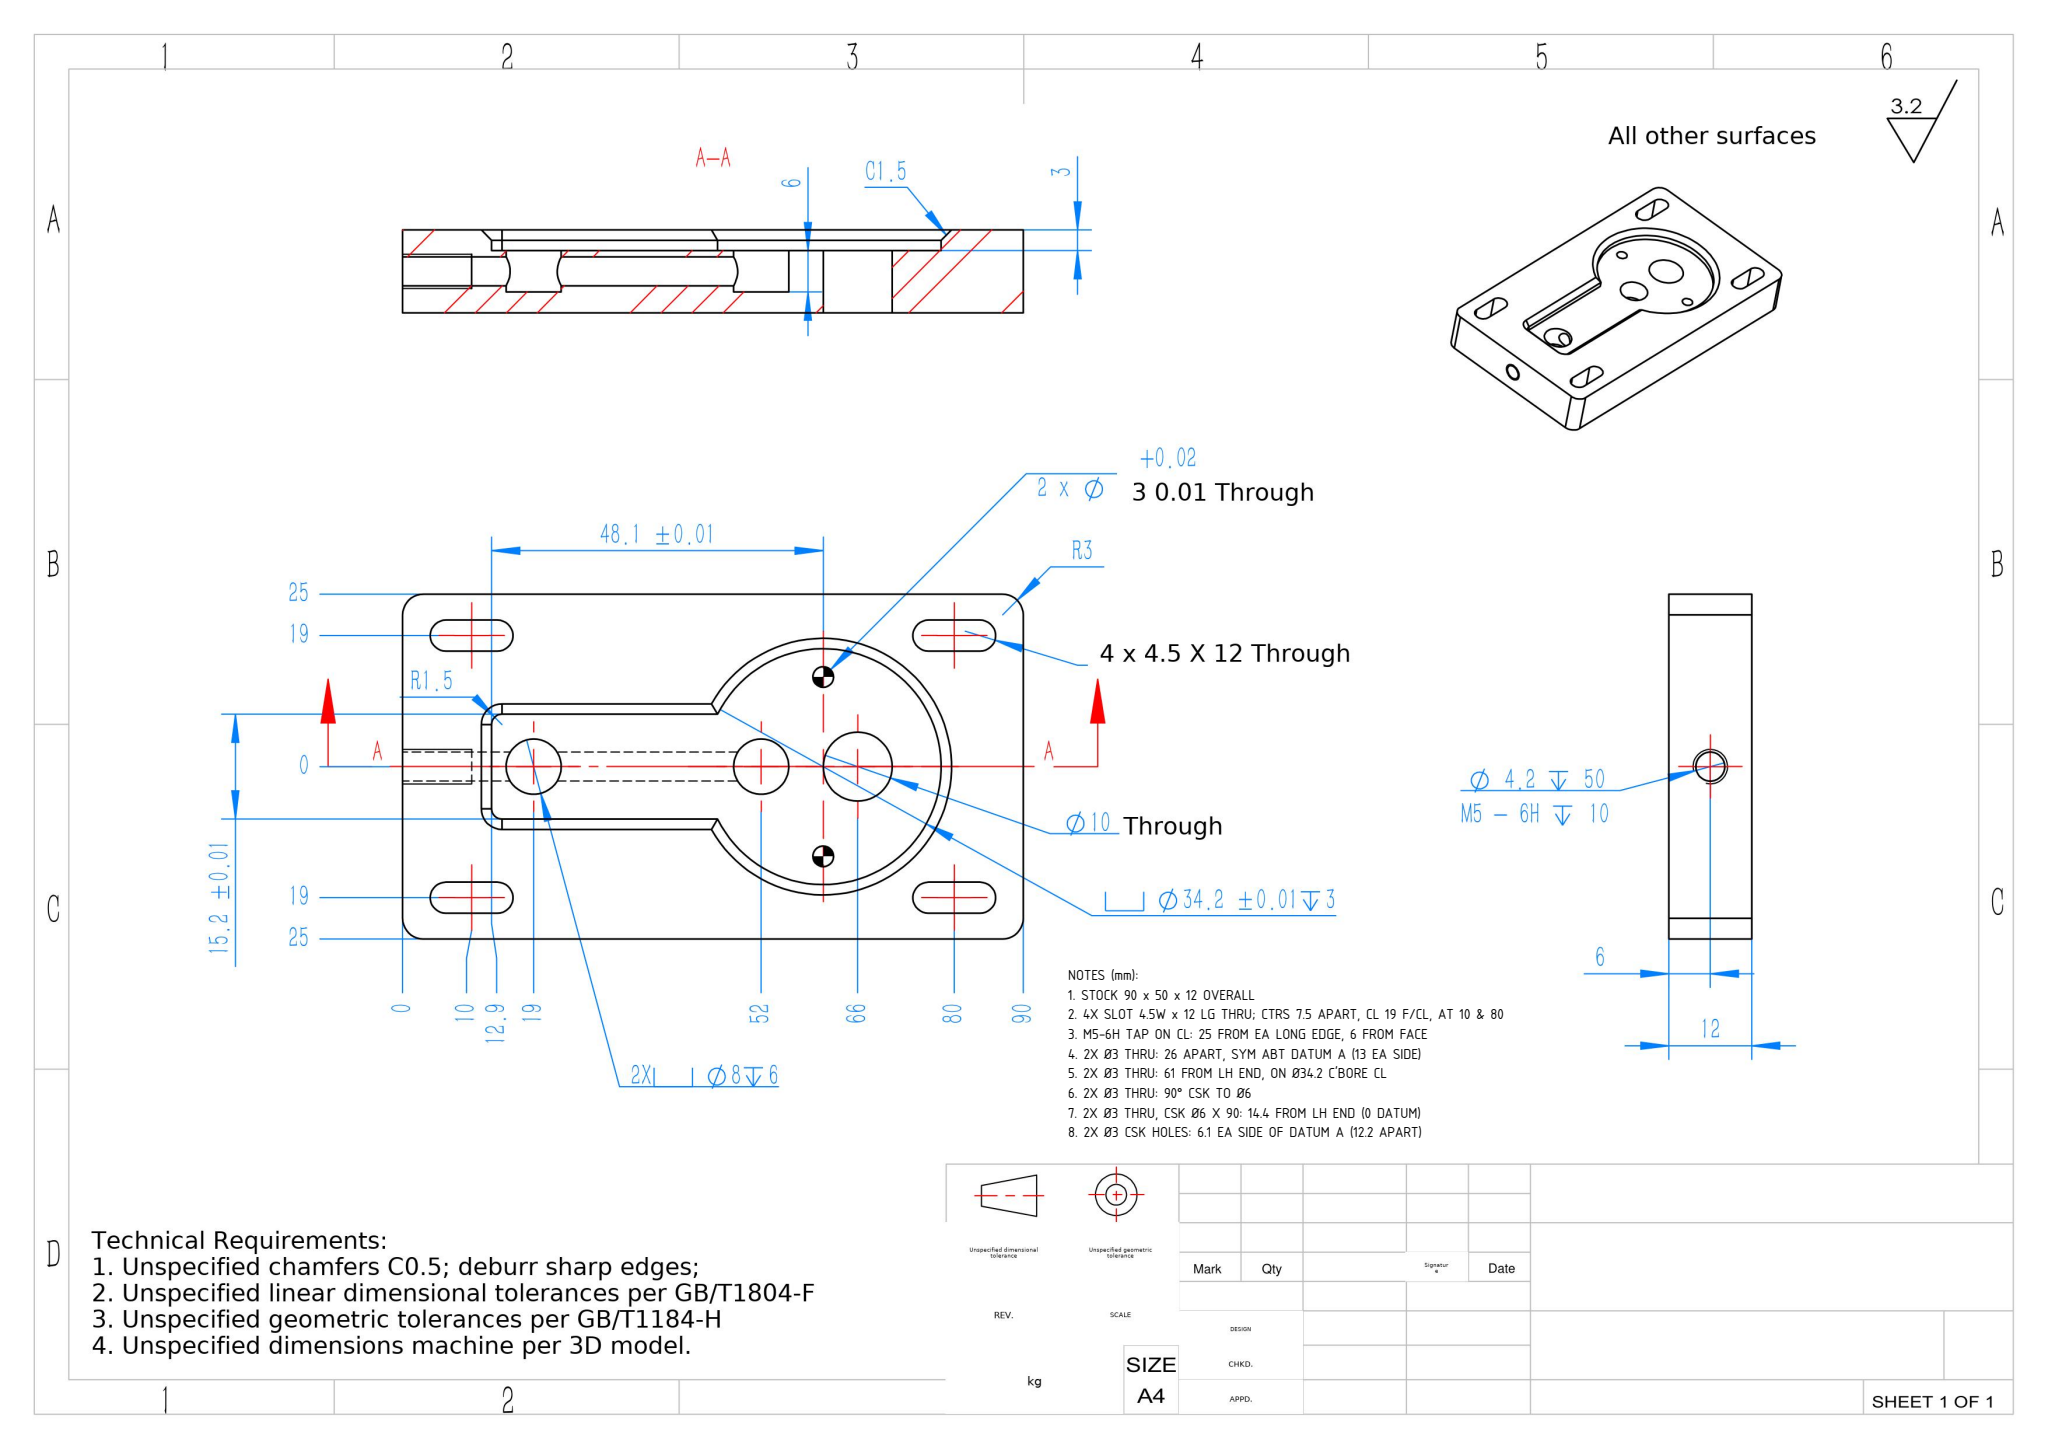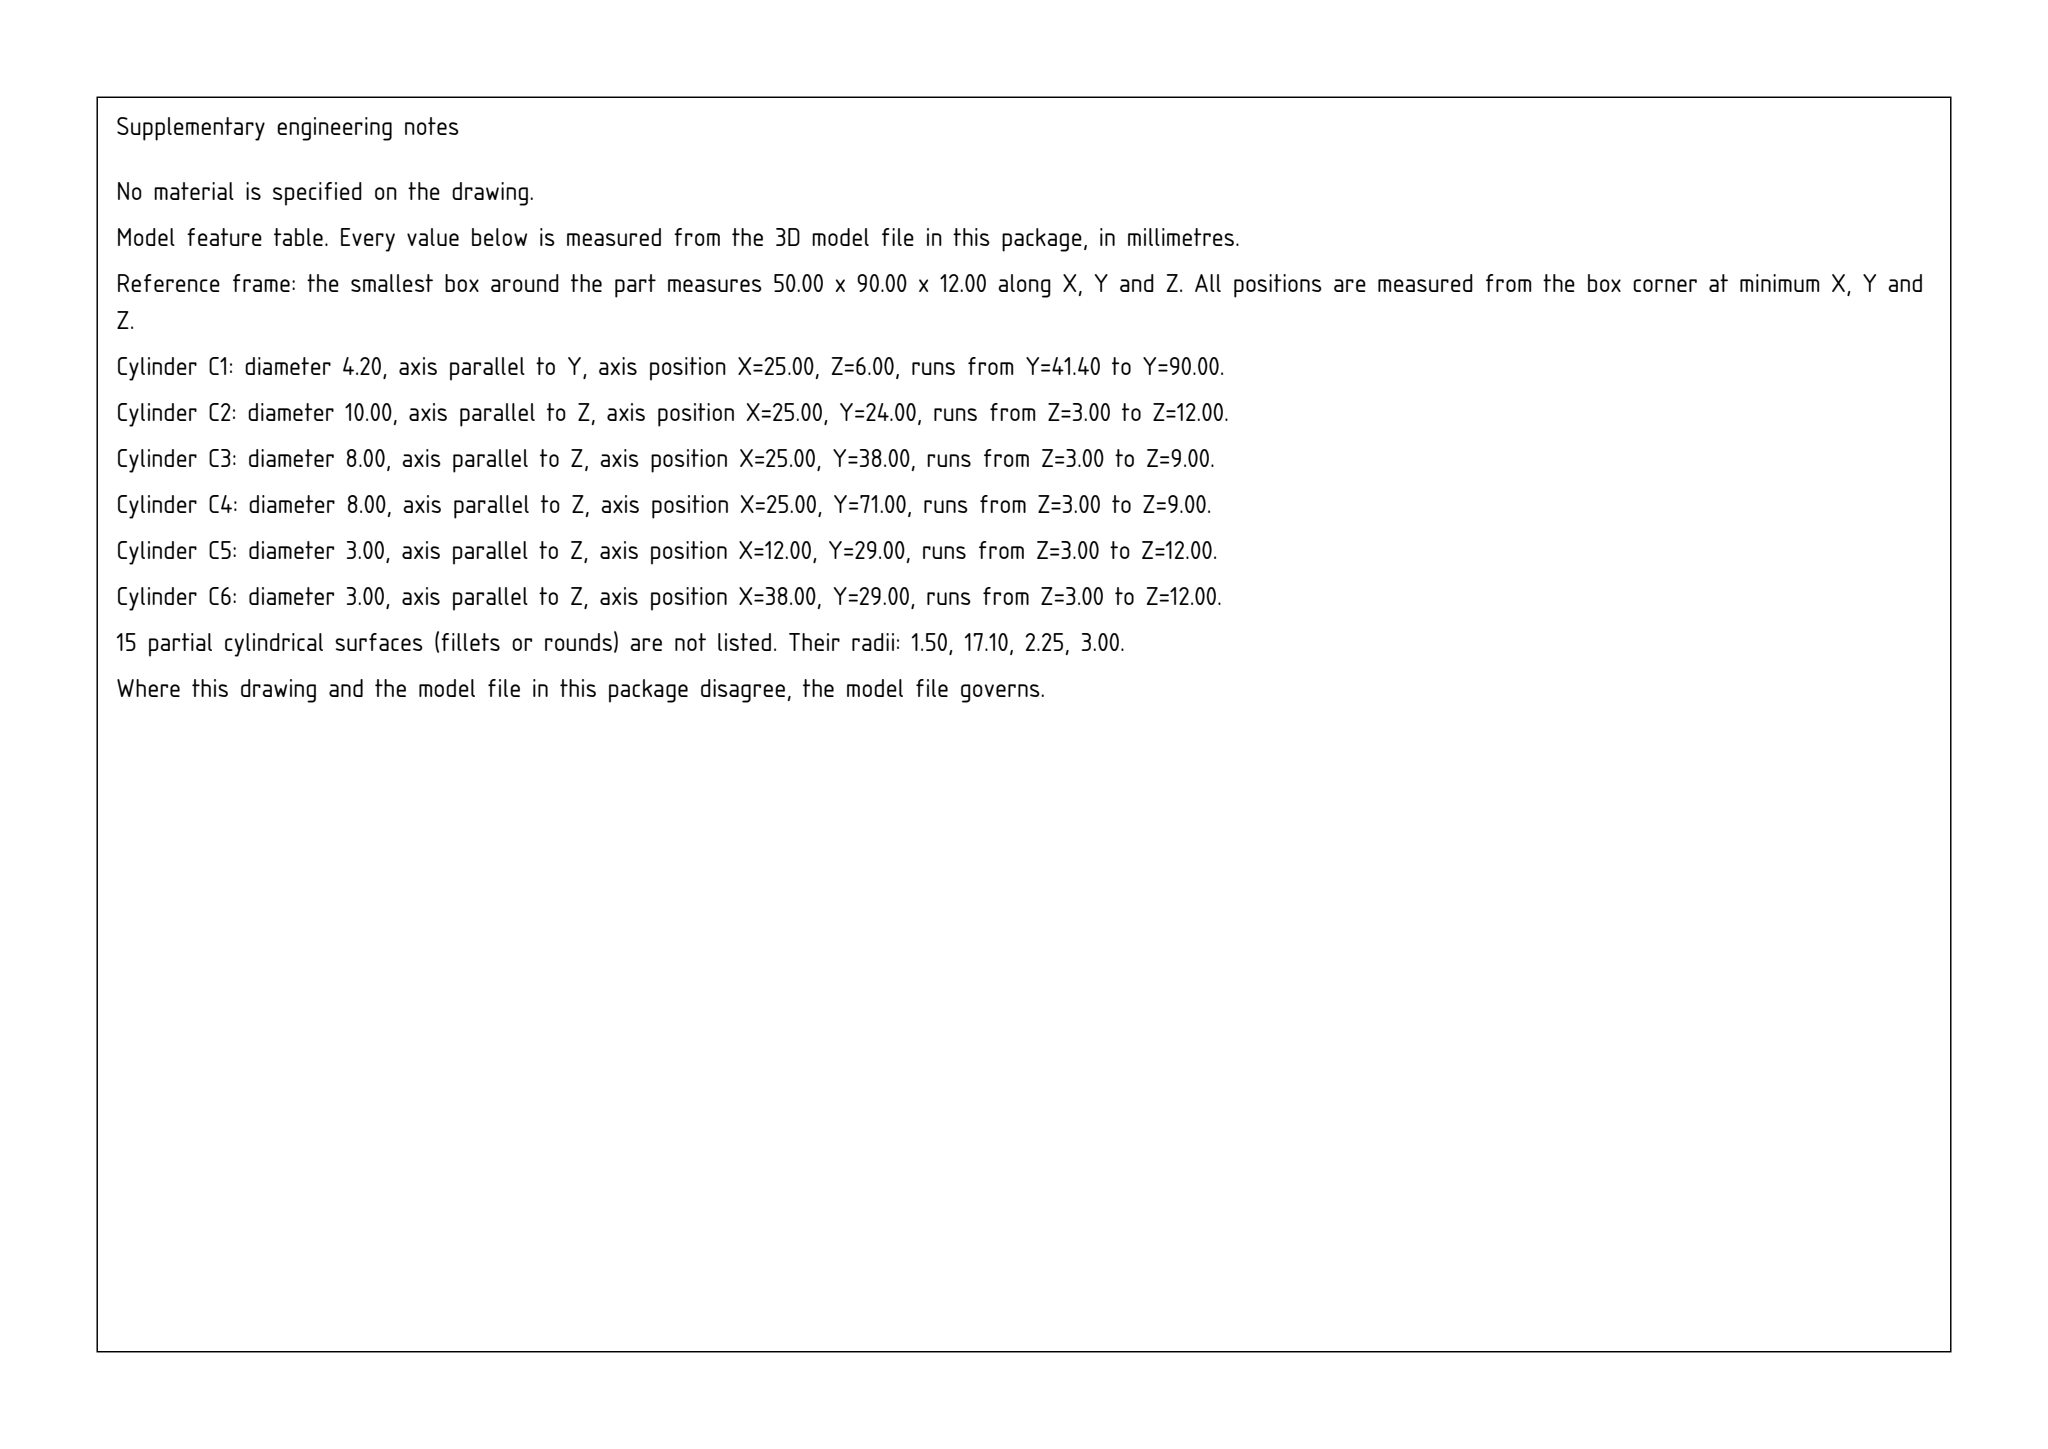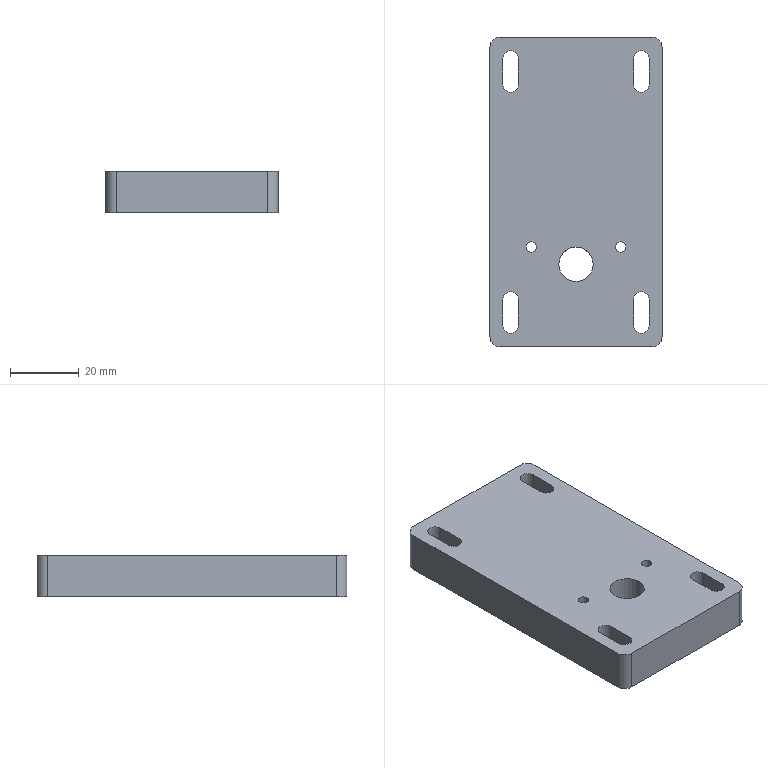Part | SolidWorks | mm | 1 solid | 59 faces | box 50 x 90 x 12 mm | volume 45137 mm3 | cylinder 31 | plane 23 | cone 5 | commonest cylinder face diameters 4.5 x8 3 x6 4.2 x4 8 x4 6 x4 34.2 x3 10 x2
Drawing notes:
STOCK 90 x 50 x 12 OVERALL | from the solid: bbox_xyz 50.0 x 90.0 x 12.0
4X SLOT 4.5W x 12 LG THRU; CTRS 7.5 APART, CL 19 F/CL, AT 10 & 80 | from the solid: Ø4.5 thru cyls (len 12) at y=6.25/13.75 and 76.25/83.75, x=6.0/44.0 => 7.5 ctr-ctr, slot ctr y=10/80, x=6 from edge = 19 from CL
M5-6H TAP ON CL: 25 FROM EA LONG EDGE, 6 FROM FACE | from the solid: Ø4.2 cyl, axis Y, at x=25.0 (of 50.0 width), z=6.0 (of 12.0 thk)
2X Ø3 THRU: 26 APART, SYM ABT DATUM A (13 EA SIDE) | from the solid: Ø3 z-holes at x=12.0 and x=38.0 (part width 50, CL x=25) => ±13, 26 apart
2X Ø3 THRU: 61 FROM LH END, ON Ø34.2 C'BORE CL | from the solid: Ø3 holes at y=29.0 and Ø34.2 c'bore at y=29.0; drawing origin at y=90 => 90-29=61
2X Ø3 THRU: 90° CSK TO Ø6 | from the solid: cones[included_angle,ref_dia]=[90.0, 6.0] qty 2, coaxial with the 2X Ø3 holes
2X Ø3 THRU, CSK Ø6 X 90: 14.4 FROM LH END (0 DATUM) | from the solid: Ø3 cyls at y=75.6 (dwg 90-75.6=14.4 from 0 end), cone 90° ref dia 6.0
2X Ø3 CSK HOLES: 6.1 EA SIDE OF DATUM A (12.2 APART) | from the solid: Ø3 cyls at x=18.9 & 31.1 vs CL x=25.0 -> ±6.1, spacing 12.2